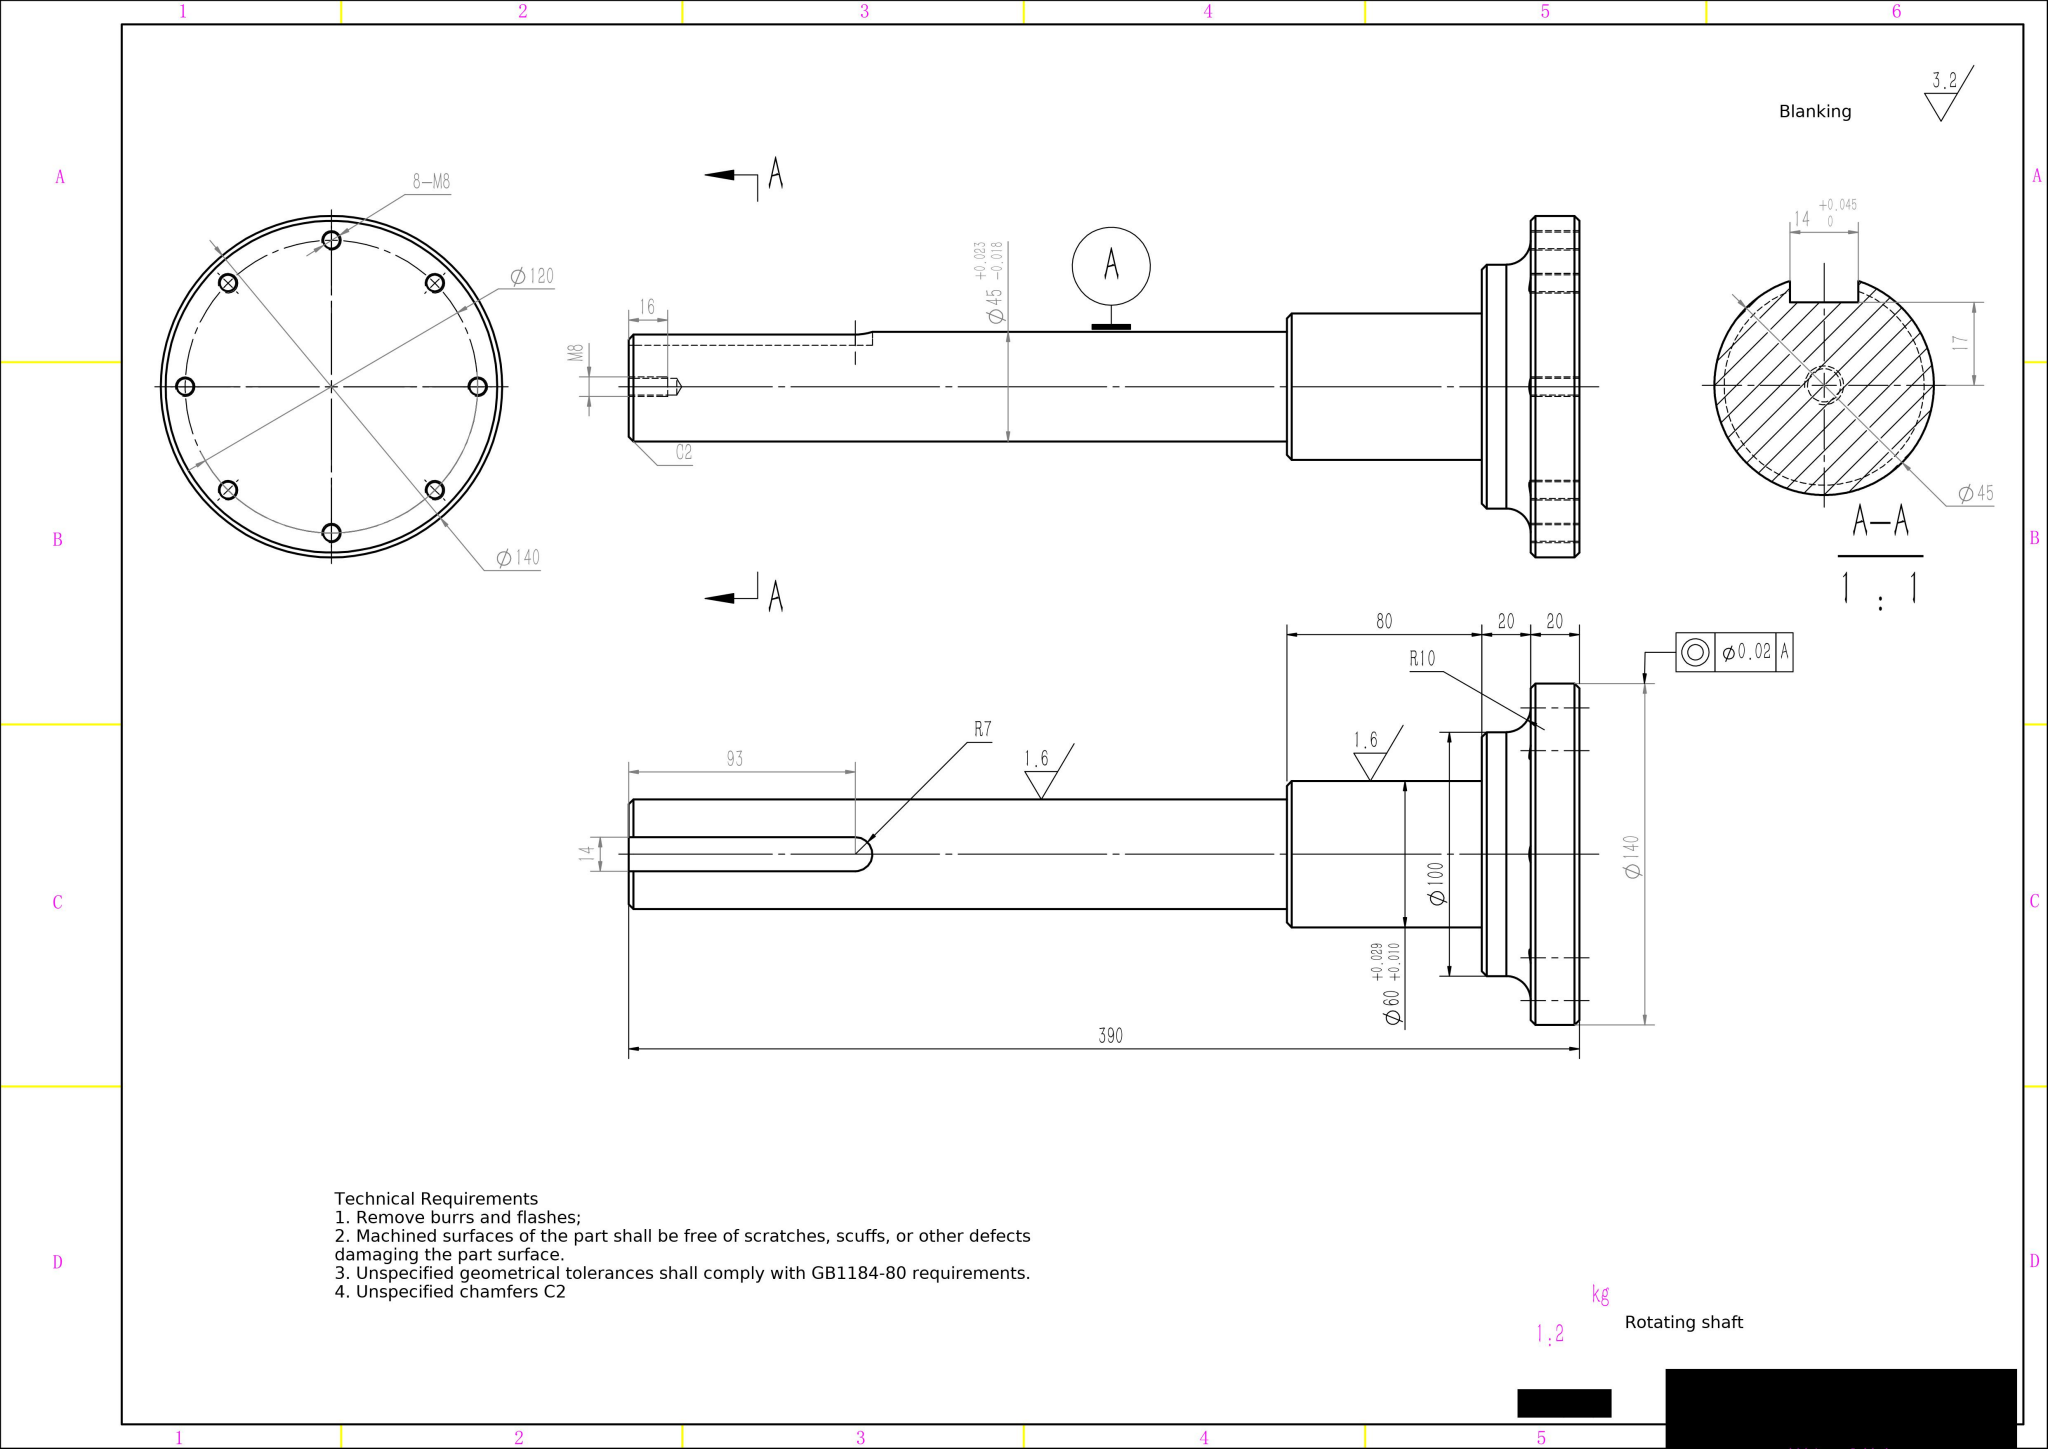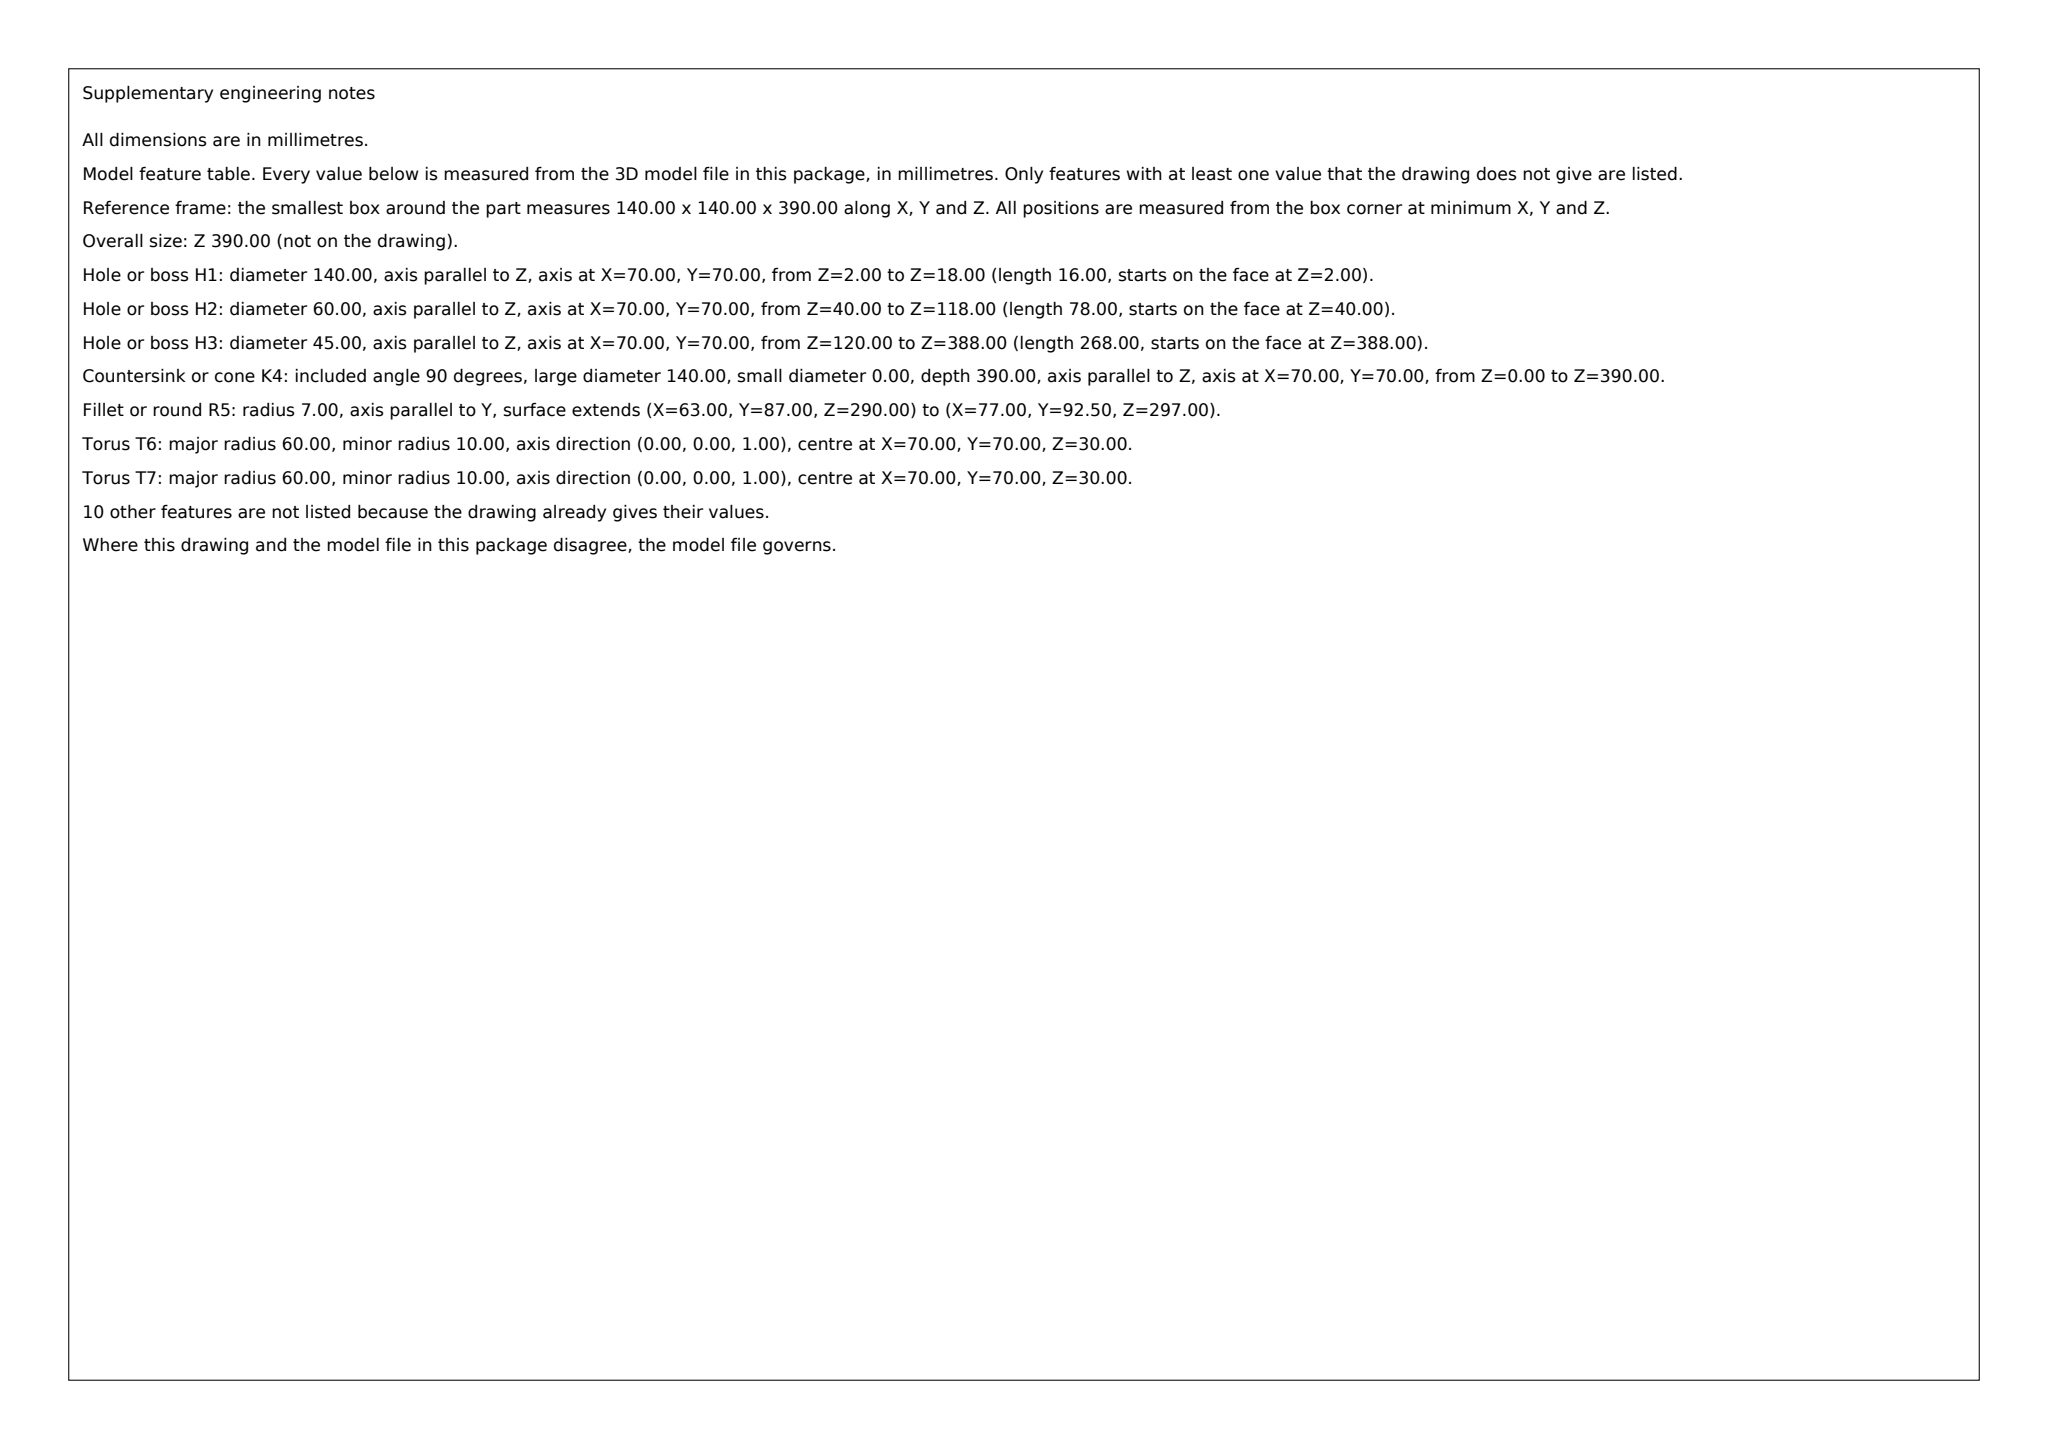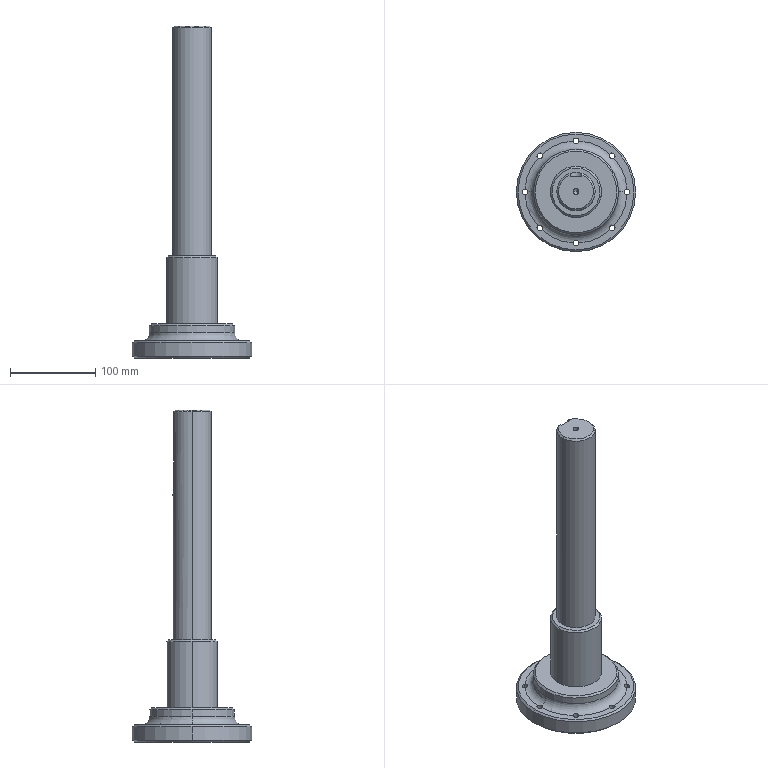Part | SolidWorks | mm | 1 solid | 50 faces | box 140 x 140 x 390 mm | volume 1110977 mm3 | cylinder 27 | cone 13 | plane 8 | torus 2 | commonest cylinder face diameters 6.8 x18 60 x2 100 x2 140 x2 45 x2 14 x1
build123d program:
from build123d import *

# Parameters (mm, degrees)
CHAMFER1_SIZE         = 2
M8_TAPPED_HOLE2_D     = 6.8
CIRPATTERN1_COUNT     = 8
CUT_EXTRUDE1_DEPTH    = 10
M8_TAPPED_HOLE1_D     = 6.8
M8_TAPPED_HOLE1_DEPTH = 19.75
M8_TAPPED_HOLE1_TIP   = 2.043


with BuildPart() as part:
    # Sketch1 → Revolve1 (revolve)
    with BuildSketch(Plane(origin=(0, 0, 0), x_dir=(1, 0, 0), z_dir=(0, 1, 0)), mode=Mode.PRIVATE) as revolve1_sk:
        with BuildLine():
            Line((0, 0), (-22.5, 0))
            Line((-22.5, 0), (-22.5, 270))
            Line((-22.5, 270), (-30, 270))
            Line((-30, 270), (-30, 350))
            Line((-30, 350), (-50, 350))
            Line((-50, 350), (-50, 360))
            ThreePointArc((-50, 360), (-52.929, 367.071), (-60, 370))
            Line((-60, 370), (-70, 370))
            Line((-70, 370), (-70, 390))
            Line((-70, 390), (0, 390))
            Line((0, 390), (0, 0))
        make_face()
    revolve(revolve1_sk.sketch.rotate(Axis((0, 0, 0), (0, 0, -1)), 180), axis=Axis((0, 0, 0), (0, 0, -1)))

    # Chamfer1
    chamfer1_edges = [part.edges().sort_by_distance(p)[0] for p in [
        (-30, 0, -270),
        (-50, 0, -350),
        (-70, 0, -370),
        (-70, 0, -390),
        (-22.5, 0, 0),
    ]]
    chamfer(chamfer1_edges, length=CHAMFER1_SIZE)

    # M8 Tapped Hole2 (through all)
    with Locations(Plane(origin=(0, 60, -390), x_dir=(-1, 0, 0), z_dir=(0, 0, -1))):
        with Locations((0, 0)):
            m8_tapped_hole2 = Hole(M8_TAPPED_HOLE2_D / 2)

    # CirPattern1: M8 Tapped Hole2 ×8 about axis
    cirpattern1_axis = Axis((0, 0, 0), (0, 0, 1))
    for i in range(1, CIRPATTERN1_COUNT):
        add(m8_tapped_hole2.rotate(cirpattern1_axis, i * 360 / CIRPATTERN1_COUNT), mode=Mode.SUBTRACT)

    # Sketch5 → Cut-Extrude1 (cut)
    with BuildSketch(Plane(origin=(0, 17, -30), x_dir=(-1, 0, 0), z_dir=(0, -1, 0))):
        with BuildLine():
            Line((7, 63), (7, -40.368))
            ThreePointArc((7, -40.368), (0, -47.368), (-7, -40.368))
            Line((-7, -40.368), (-7, 63))
            ThreePointArc((-7, 63), (0, 70), (7, 63))
        make_face()
    extrude(amount=-CUT_EXTRUDE1_DEPTH, mode=Mode.SUBTRACT)

    # M8 Tapped Hole1
    with Locations(Plane.XY):
        with Locations((0, 0)):
            Hole(M8_TAPPED_HOLE1_D / 2, depth=M8_TAPPED_HOLE1_DEPTH)
            with Locations((0, 0, -(M8_TAPPED_HOLE1_DEPTH + M8_TAPPED_HOLE1_TIP / 2))):  # 118° drill point
                Cone(0, M8_TAPPED_HOLE1_D / 2, M8_TAPPED_HOLE1_TIP, mode=Mode.SUBTRACT)


solid = part.part